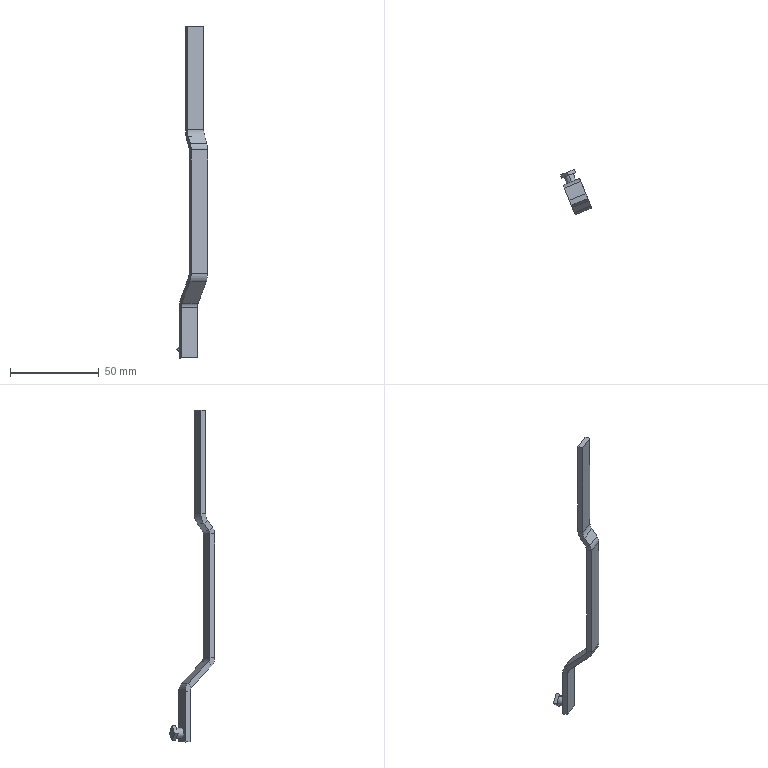Component | SolidWorks | RightDoorAssembly-1_LinkRodLock-1_Lock-1_LowerRod-1 | 1 solid | 46 faces | volume 6013 mm3 | plane 36 | cylinder 10 | commonest cylinder face diameters 12 x4 6 x3 5.5 x2 18 x1